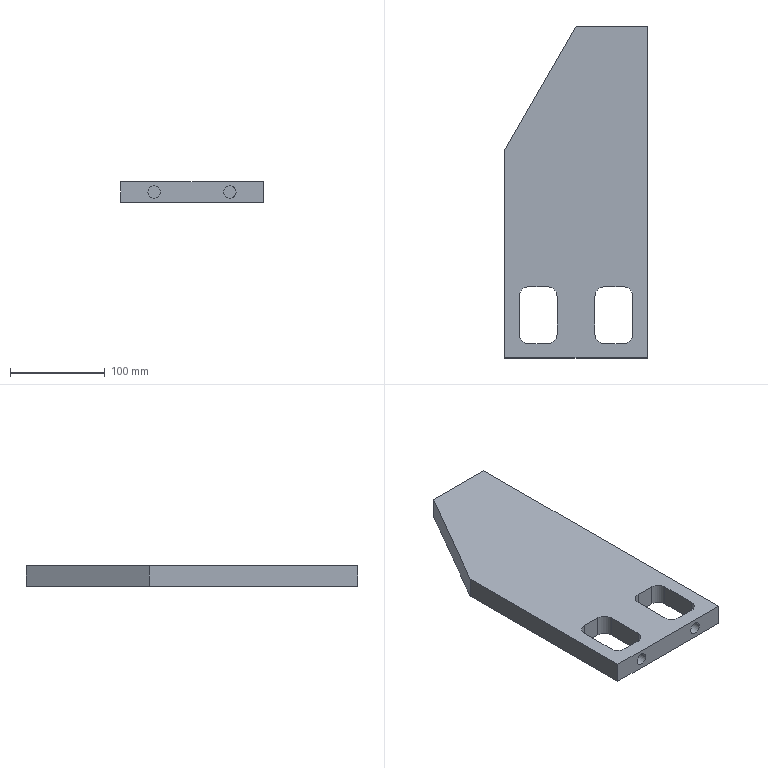Component | SolidWorks | Assembly2-1_SideReinforcementPlate-1 | 1 solid | 38 faces | box 150 x 350 x 22 mm | volume 935692 mm3 | cylinder 19 | plane 15 | cone 4 | commonest cylinder face diameters 20 x9 10.2 x6 13 x4
build123d program:
from build123d import *

# Parameters (mm, degrees)
SKETCH1_W              = 22
SKETCH1_H              = 350
BOSS_EXTRUDE1_DEPTH    = 150
CUT_EXTRUDE1_DEPTH     = 382.424
CUT_EXTRUDE2_DEPTH     = 382.424
SKETCH4_R              = 6.5
CUT_EXTRUDE3_DEPTH     = 20
M12_TAPPED_HOLE1_D     = 10.2
M12_TAPPED_HOLE1_DEPTH = 29.25
M12_TAPPED_HOLE1_TIP   = 3.064


with BuildPart() as part:
    # Sketch1 → Boss-Extrude1 (new body)
    with BuildSketch(Plane.XY):
        with Locations((11, 175)):
            Rectangle(SKETCH1_W, SKETCH1_H)
    extrude(amount=BOSS_EXTRUDE1_DEPTH)

    # Sketch2 → Cut-Extrude1 (cut, through all)
    with BuildSketch(Plane(origin=(22, 0, 0), x_dir=(0, 0, -1), z_dir=(1, 0, 0))):
        with BuildLine():
            Line((-125, 75), (-105, 75))
            ThreePointArc((-105, 75), (-97.929, 72.071), (-95, 65))
            Line((-95, 65), (-95, 25))
            ThreePointArc((-95, 25), (-97.929, 17.929), (-105, 15))
            Line((-105, 15), (-125, 15))
            ThreePointArc((-125, 15), (-132.071, 17.929), (-135, 25))
            Line((-135, 25), (-135, 65))
            ThreePointArc((-135, 65), (-132.071, 72.071), (-125, 75))
        make_face()
        with BuildLine():
            Line((-55, 65), (-55, 25))
            ThreePointArc((-55, 25), (-52.071, 17.929), (-45, 15))
            Line((-45, 15), (-25, 15))
            ThreePointArc((-25, 15), (-17.929, 17.929), (-15, 25))
            Line((-15, 25), (-15, 65))
            ThreePointArc((-15, 65), (-17.929, 72.071), (-25, 75))
            Line((-25, 75), (-45, 75))
            ThreePointArc((-45, 75), (-52.071, 72.071), (-55, 65))
        make_face()
    extrude(amount=-CUT_EXTRUDE1_DEPTH, mode=Mode.SUBTRACT)

    # Sketch3 → Cut-Extrude2 (cut, through all)
    with BuildSketch(Plane.ZY):
        Polygon((75, 350), (0, 220.096), (0, 350), align=None)
    extrude(amount=-CUT_EXTRUDE2_DEPTH, mode=Mode.SUBTRACT)

    # Sketch4 → Cut-Extrude3 (cut)
    with BuildSketch(Plane.XZ):
        with Locations(Location((11, 115, 0), (0, 0, 270))):
            Circle(SKETCH4_R)
        with Locations((11, 35)):
            Circle(SKETCH4_R)
    extrude(amount=-CUT_EXTRUDE3_DEPTH, mode=Mode.SUBTRACT)

    # M12 Tapped Hole1
    with Locations(Plane(origin=(11, 20, 150), x_dir=(1, 0, 0), z_dir=(0, 0, 1))):
        with Locations((0, 0), (0, 155), (0, 310)):
            Hole(M12_TAPPED_HOLE1_D / 2, depth=M12_TAPPED_HOLE1_DEPTH)
            with Locations((0, 0, -(M12_TAPPED_HOLE1_DEPTH + M12_TAPPED_HOLE1_TIP / 2))):  # 118° drill point
                Cone(0, M12_TAPPED_HOLE1_D / 2, M12_TAPPED_HOLE1_TIP, mode=Mode.SUBTRACT)


solid = part.part

# Placed as in the assembly
solid = solid.moved(Location((-803.02, -324.181, 62), (0, 90, 0)))